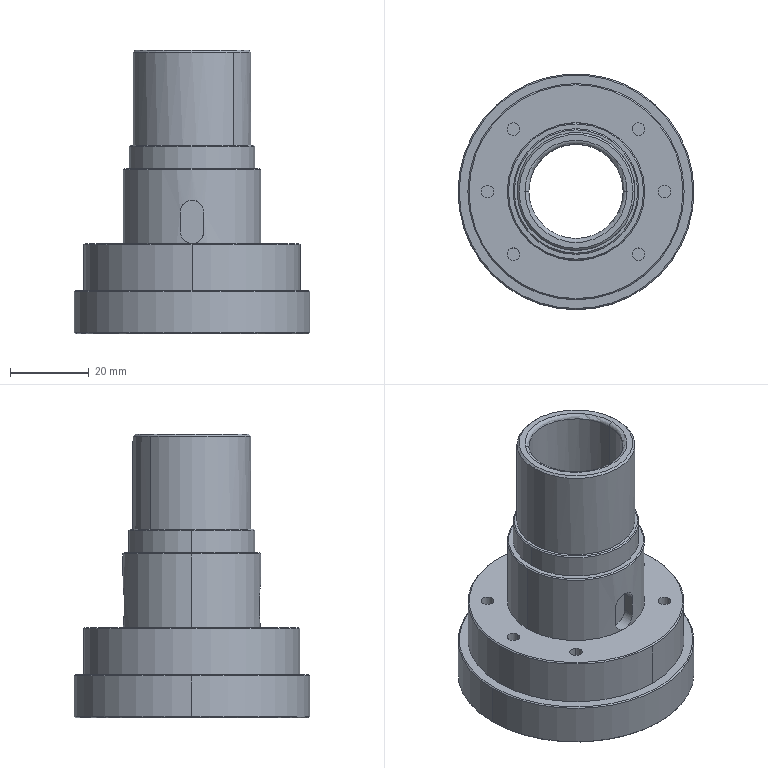CAM job | Mastercam | mm | 3 operations | part box 60 x 60 x 72.2
1. Drill/Counterbore | 17 - 6 倒角刀
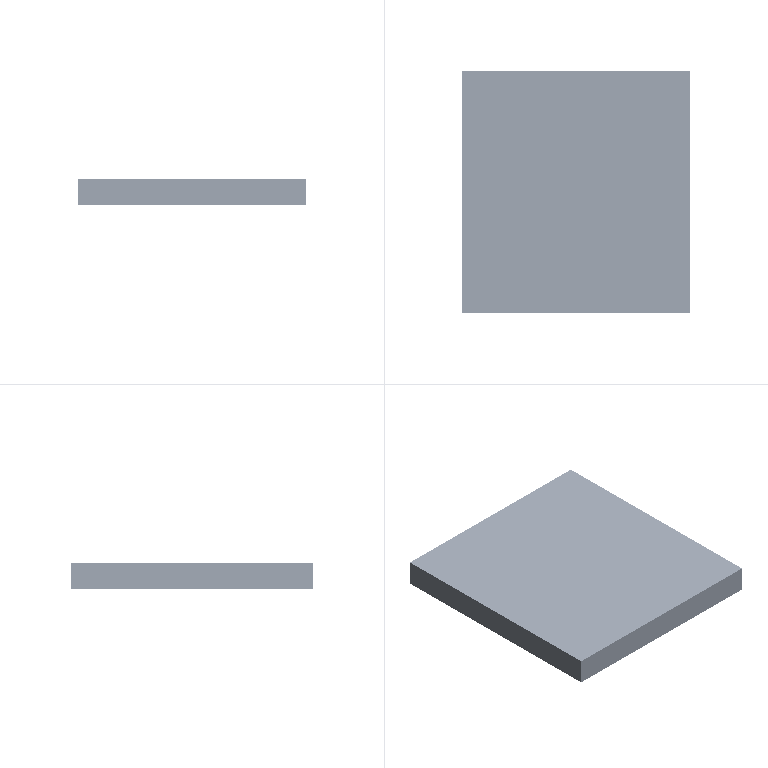2. Contour (Ramp) | 4 - 4 平铣刀
3. Contour (Ramp) | 1 - 4 平铣刀